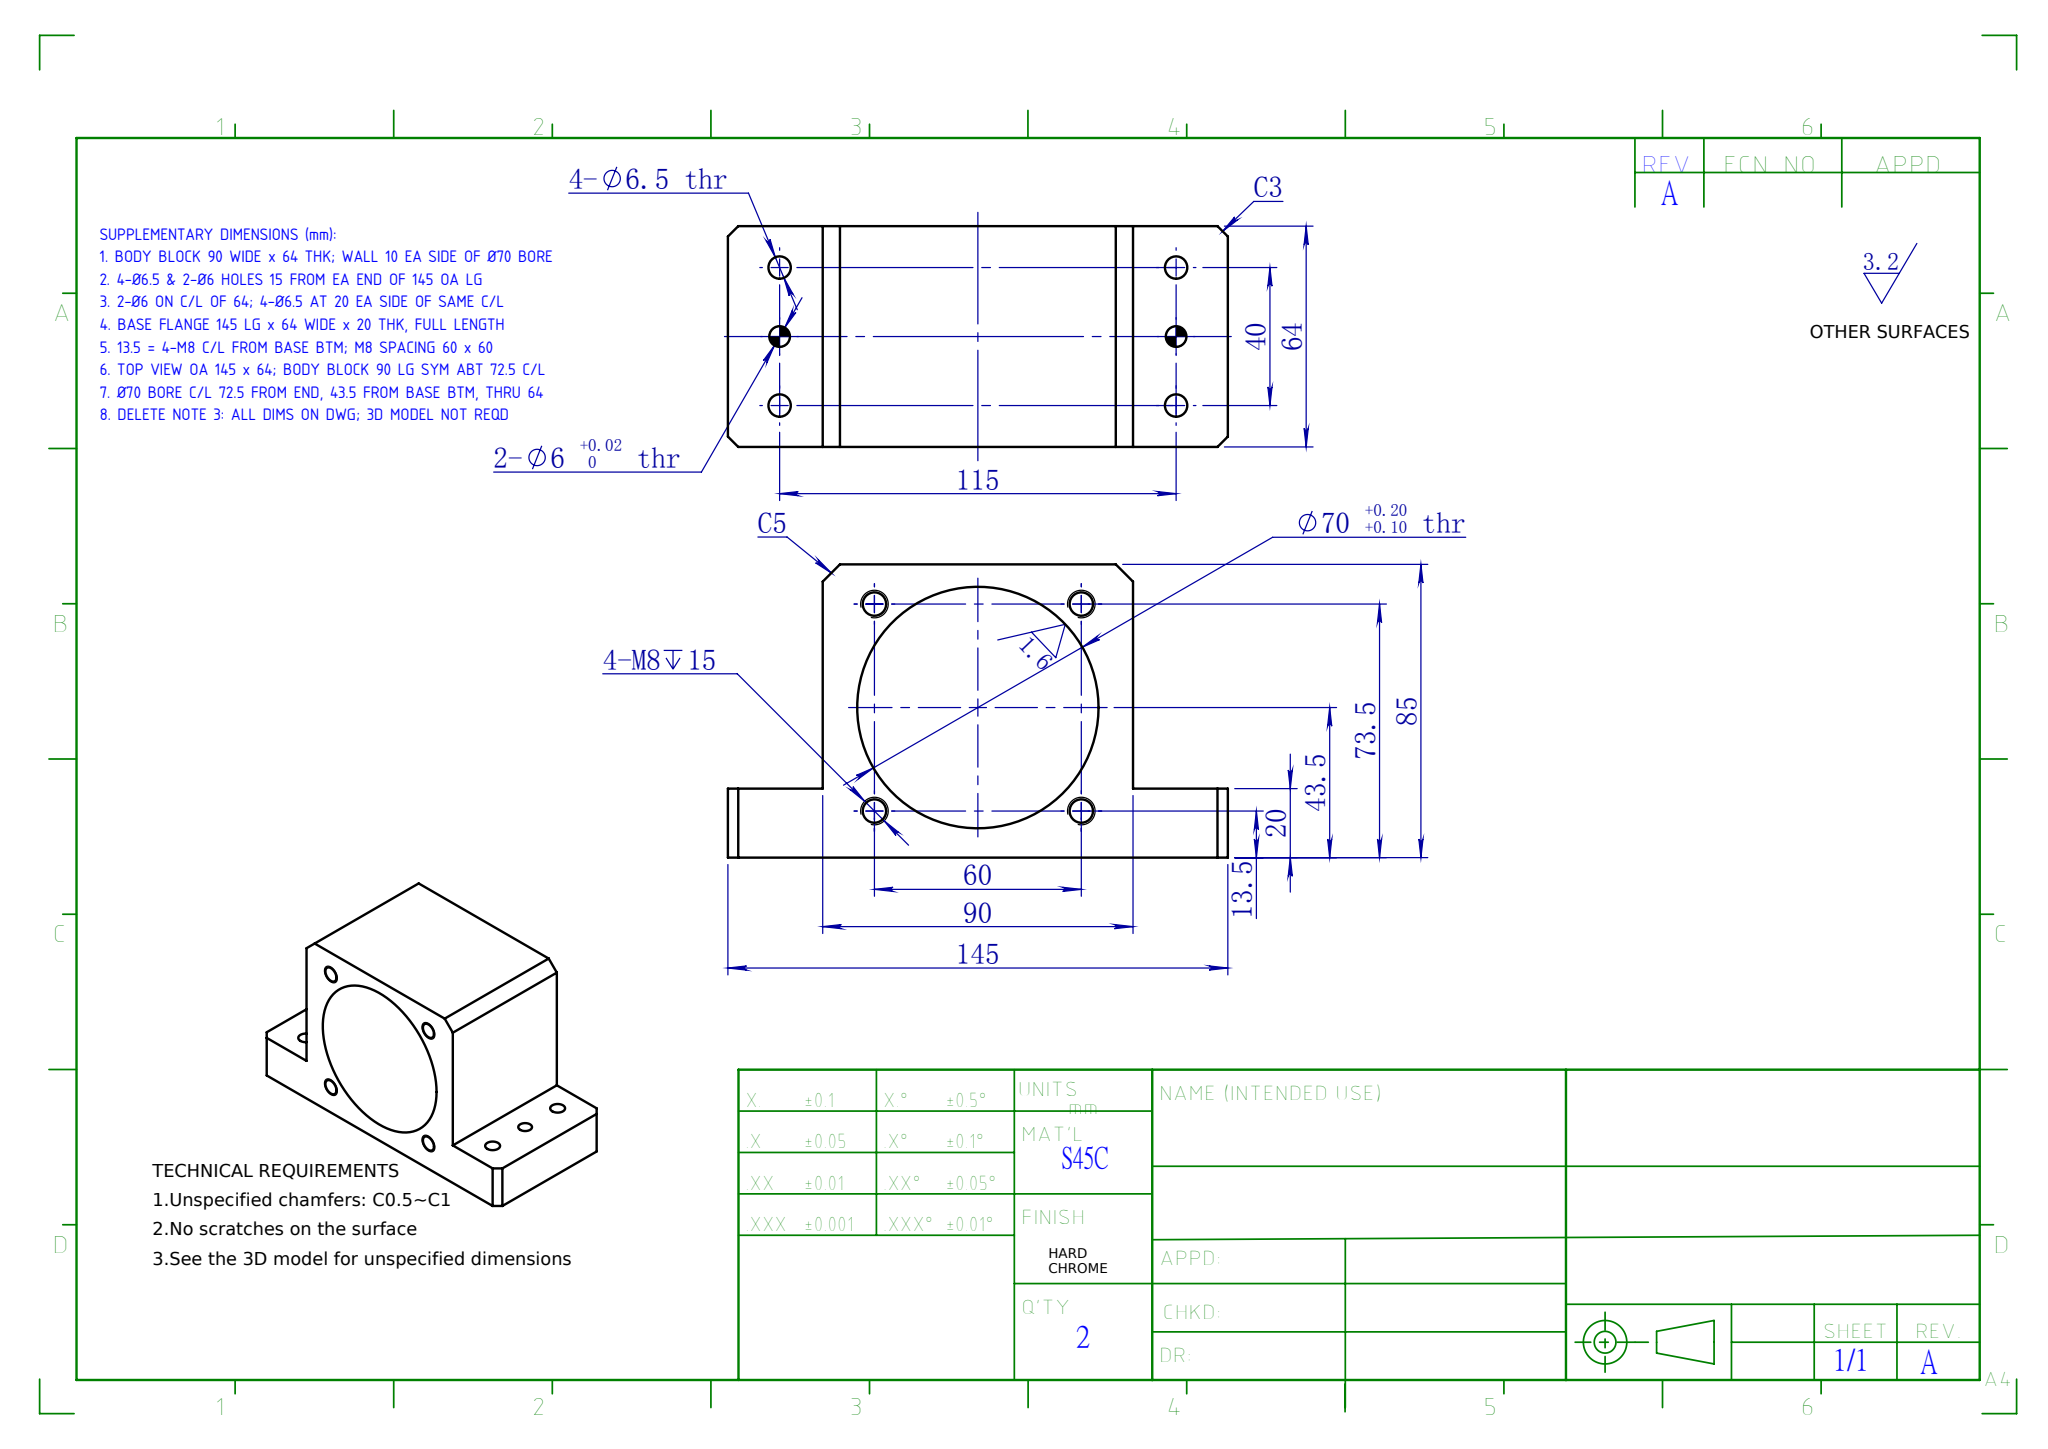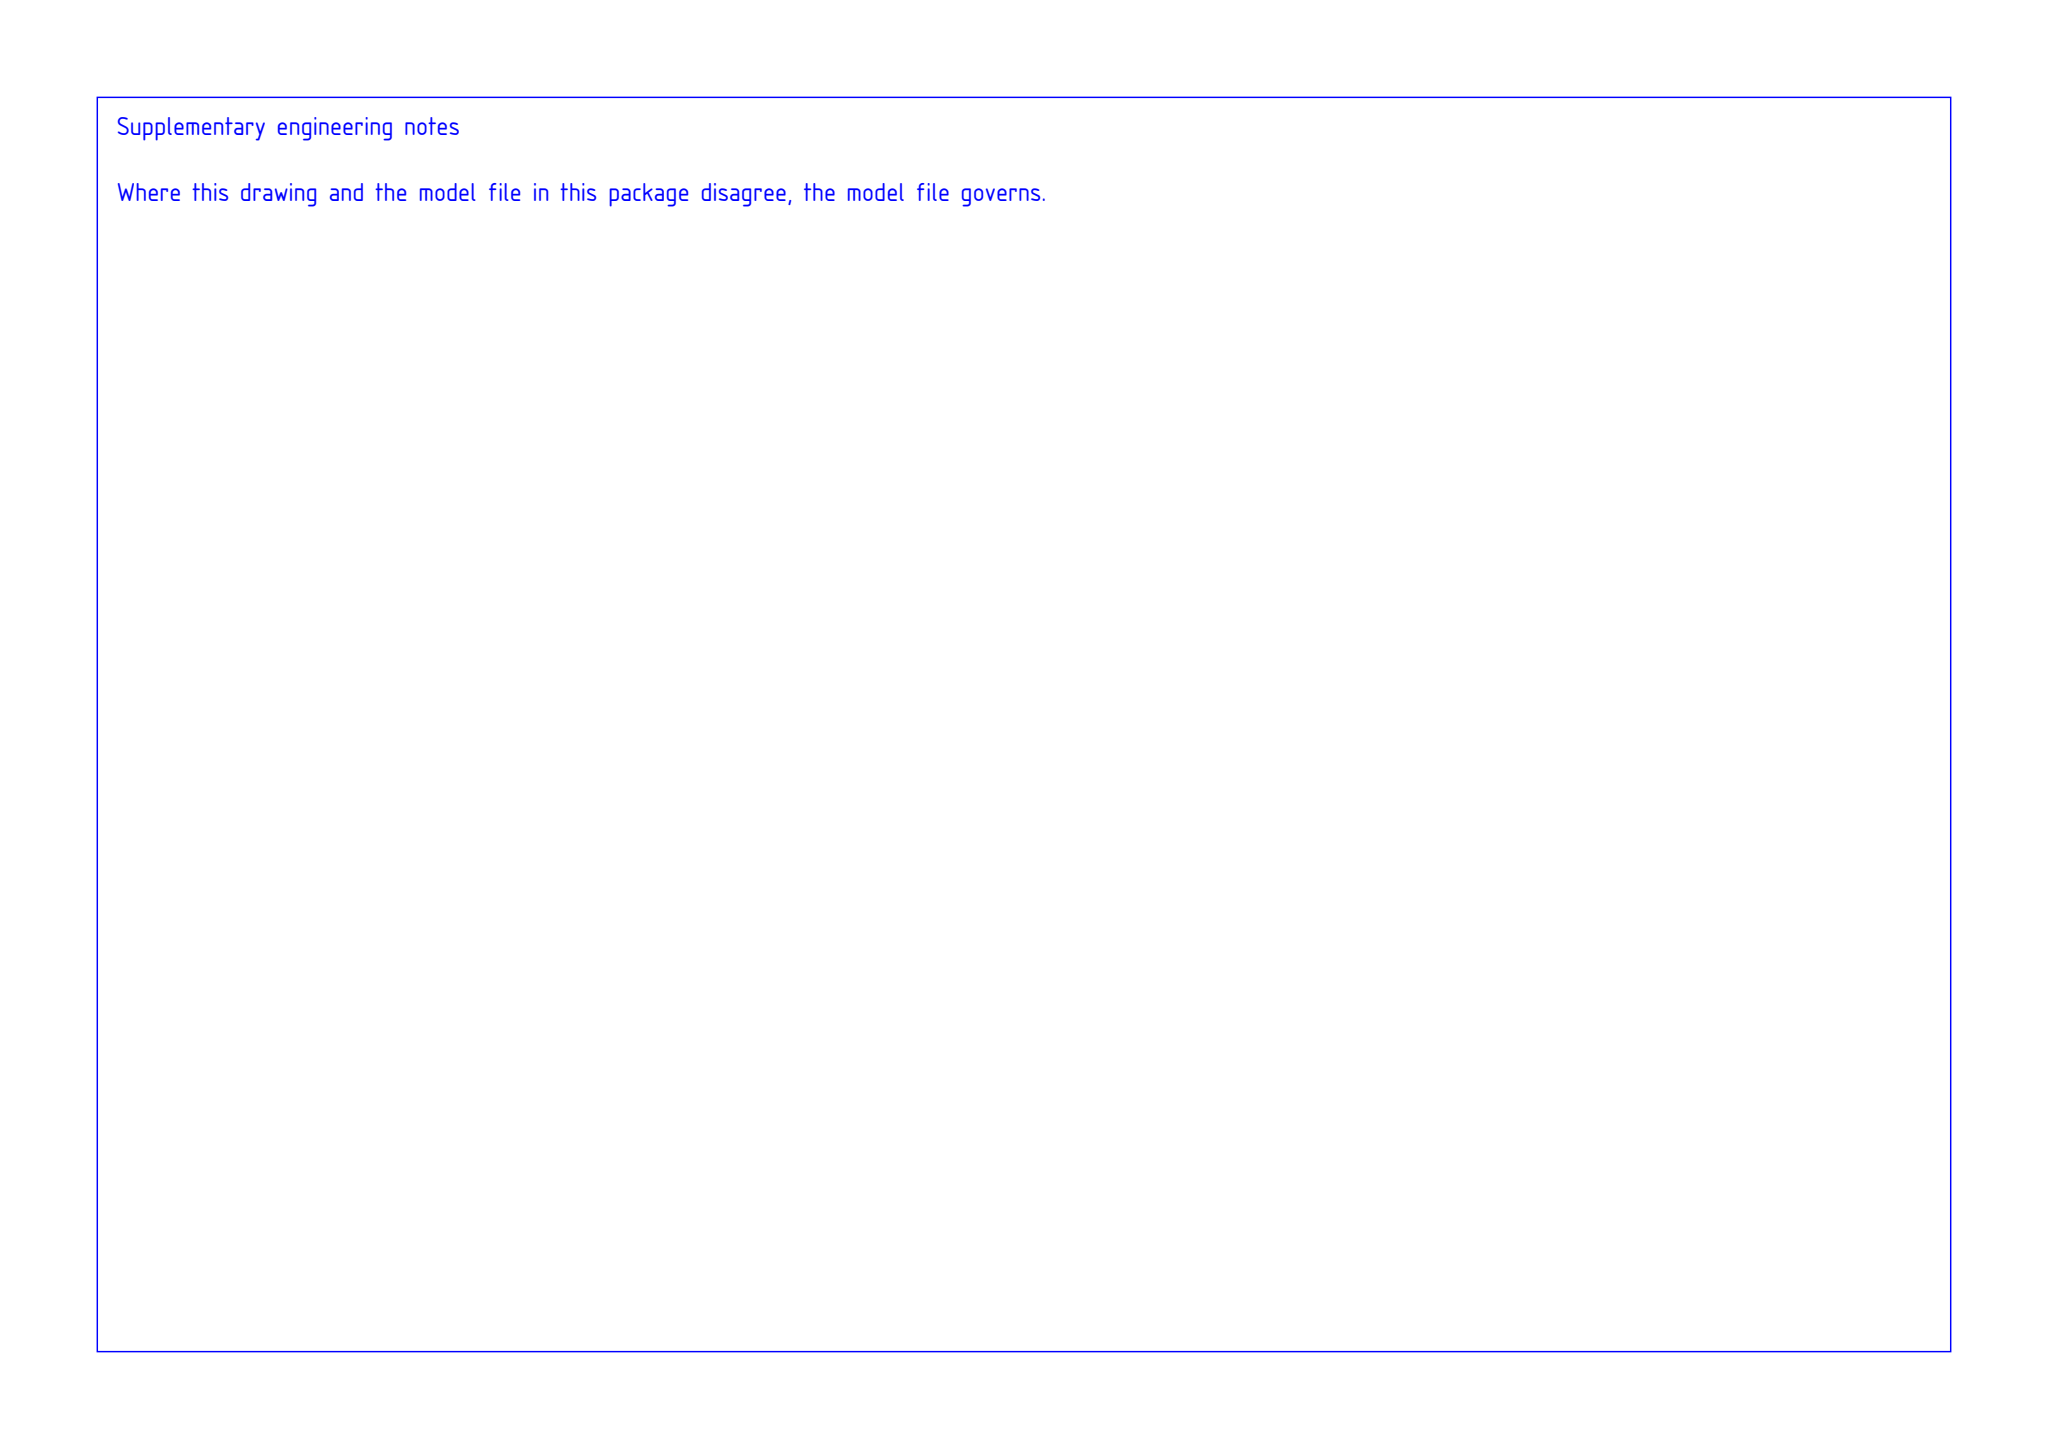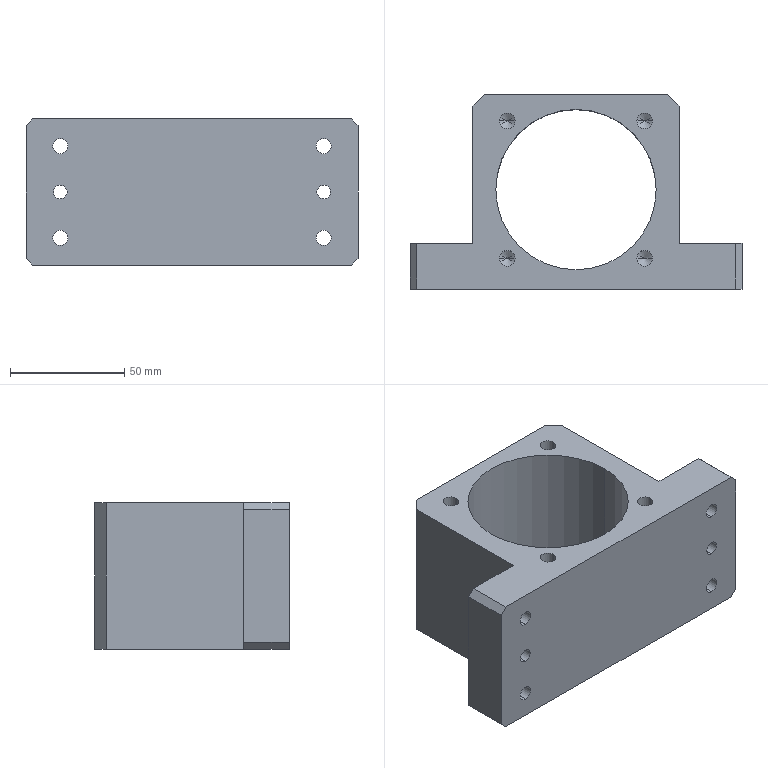Part | SolidWorks | mm | 1 solid | 46 faces | box 145 x 85 x 64 mm | volume 305676 mm3 | cylinder 22 | plane 16 | cone 8 | commonest cylinder face diameters 6.8 x8 6.5 x8 6 x4 70 x2
build123d program:
from build123d import *

# Parameters (mm, degrees)
SKETCH1_W             = 90
SKETCH1_H             = 64
BOSS_EXTRUDE1_DEPTH   = 85
SKETCH1_2_R           = 35
CUT_EXTRUDE1_DEPTH    = 116.525
SKETCH2_W             = 64
SKETCH2_H             = 20
BOSS_EXTRUDE1_2_DEPTH = 27.5
SKETCH3_R             = 3.25
CUT_EXTRUDE2_DEPTH    = 103.495
CHAMFER1_SIZE         = 5
M8_TAPPED_HOLE1_D     = 6.8
M8_TAPPED_HOLE1_DEPTH = 15
M8_TAPPED_HOLE1_TIP   = 2.043
CHAMFER2_SIZE         = 3
SKETCH2_2_R           = 3
CUT_EXTRUDE1_2_DEPTH  = 103.495


with BuildPart() as part:
    # Sketch1 → Boss-Extrude1 (new body)
    with BuildSketch(Plane(origin=(0, 0, 0), x_dir=(1, 0, 0), z_dir=(0, 1, 0))):
        Rectangle(SKETCH1_W, SKETCH1_H)
    extrude(amount=BOSS_EXTRUDE1_DEPTH)

    # Sketch1_2 → Cut-Extrude1 (cut, through all)
    with BuildSketch(Plane.XY.offset(32)):
        with Locations((0, 43.5)):
            Circle(SKETCH1_2_R)
    extrude(amount=-CUT_EXTRUDE1_DEPTH, mode=Mode.SUBTRACT)

    # Sketch2 → Boss-Extrude1_2 (add)
    with BuildSketch(Plane.ZY.offset(45)):
        with Locations((0, 10)):
            Rectangle(SKETCH2_W, SKETCH2_H)
    boss_extrude1_2 = extrude(amount=BOSS_EXTRUDE1_2_DEPTH)

    # Sketch3 → Cut-Extrude2 (cut, through all)
    with BuildSketch(Plane(origin=(0, 20, 0), x_dir=(1, 0, 0), z_dir=(0, 1, 0))):
        with Locations(Location((-57.5, 20, 0), (0, 0, 270))):
            Circle(SKETCH3_R)
        with Locations(Location((-57.5, -20, 0), (0, 0, 270))):
            Circle(SKETCH3_R)
    cut_extrude2 = extrude(amount=-CUT_EXTRUDE2_DEPTH, mode=Mode.SUBTRACT)

    # Mirror1: Boss-Extrude1_2, Cut-Extrude2 across plane
    add(boss_extrude1_2.mirror(Plane(origin=(0, 0, 0), x_dir=(0, 0, 1), z_dir=(1, 0, 0))))
    add(cut_extrude2.mirror(Plane(origin=(0, 0, 0), x_dir=(0, 0, 1), z_dir=(1, 0, 0))), mode=Mode.SUBTRACT)

    # Chamfer1
    chamfer1_edges = [part.edges().sort_by_distance(p)[0] for p in [
        (45, 85, 0),
        (-45, 85, 0),
    ]]
    chamfer(chamfer1_edges, length=CHAMFER1_SIZE)

    # M8 Tapped Hole1
    with Locations(Plane.XY.offset(32)):
        with Locations((30, 73.5), (30, 13.5), (-30, 73.5), (-30, 13.5)):
            Hole(M8_TAPPED_HOLE1_D / 2, depth=M8_TAPPED_HOLE1_DEPTH)
            with Locations((0, 0, -(M8_TAPPED_HOLE1_DEPTH + M8_TAPPED_HOLE1_TIP / 2))):  # 118° drill point
                Cone(0, M8_TAPPED_HOLE1_D / 2, M8_TAPPED_HOLE1_TIP, mode=Mode.SUBTRACT)

    # Chamfer2
    chamfer2_edges = [part.edges().sort_by_distance(p)[0] for p in [
        (72.5, 10, -32),
        (72.5, 10, 32),
        (-72.5, 10, 32),
        (-72.5, 10, -32),
    ]]
    chamfer(chamfer2_edges, length=CHAMFER2_SIZE)

    # Sketch2_2 → Cut-Extrude1_2 (cut, through all)
    with BuildSketch(Plane(origin=(0, 20, 0), x_dir=(1, 0, 0), z_dir=(0, 1, 0))):
        with Locations(Location((-57.5, 0, 0), (0, 0, 270))):
            Circle(SKETCH2_2_R)
        with Locations(Location((57.5, 0, 0), (0, 0, 270))):
            Circle(SKETCH2_2_R)
    extrude(amount=-CUT_EXTRUDE1_2_DEPTH, mode=Mode.SUBTRACT)


solid = part.part